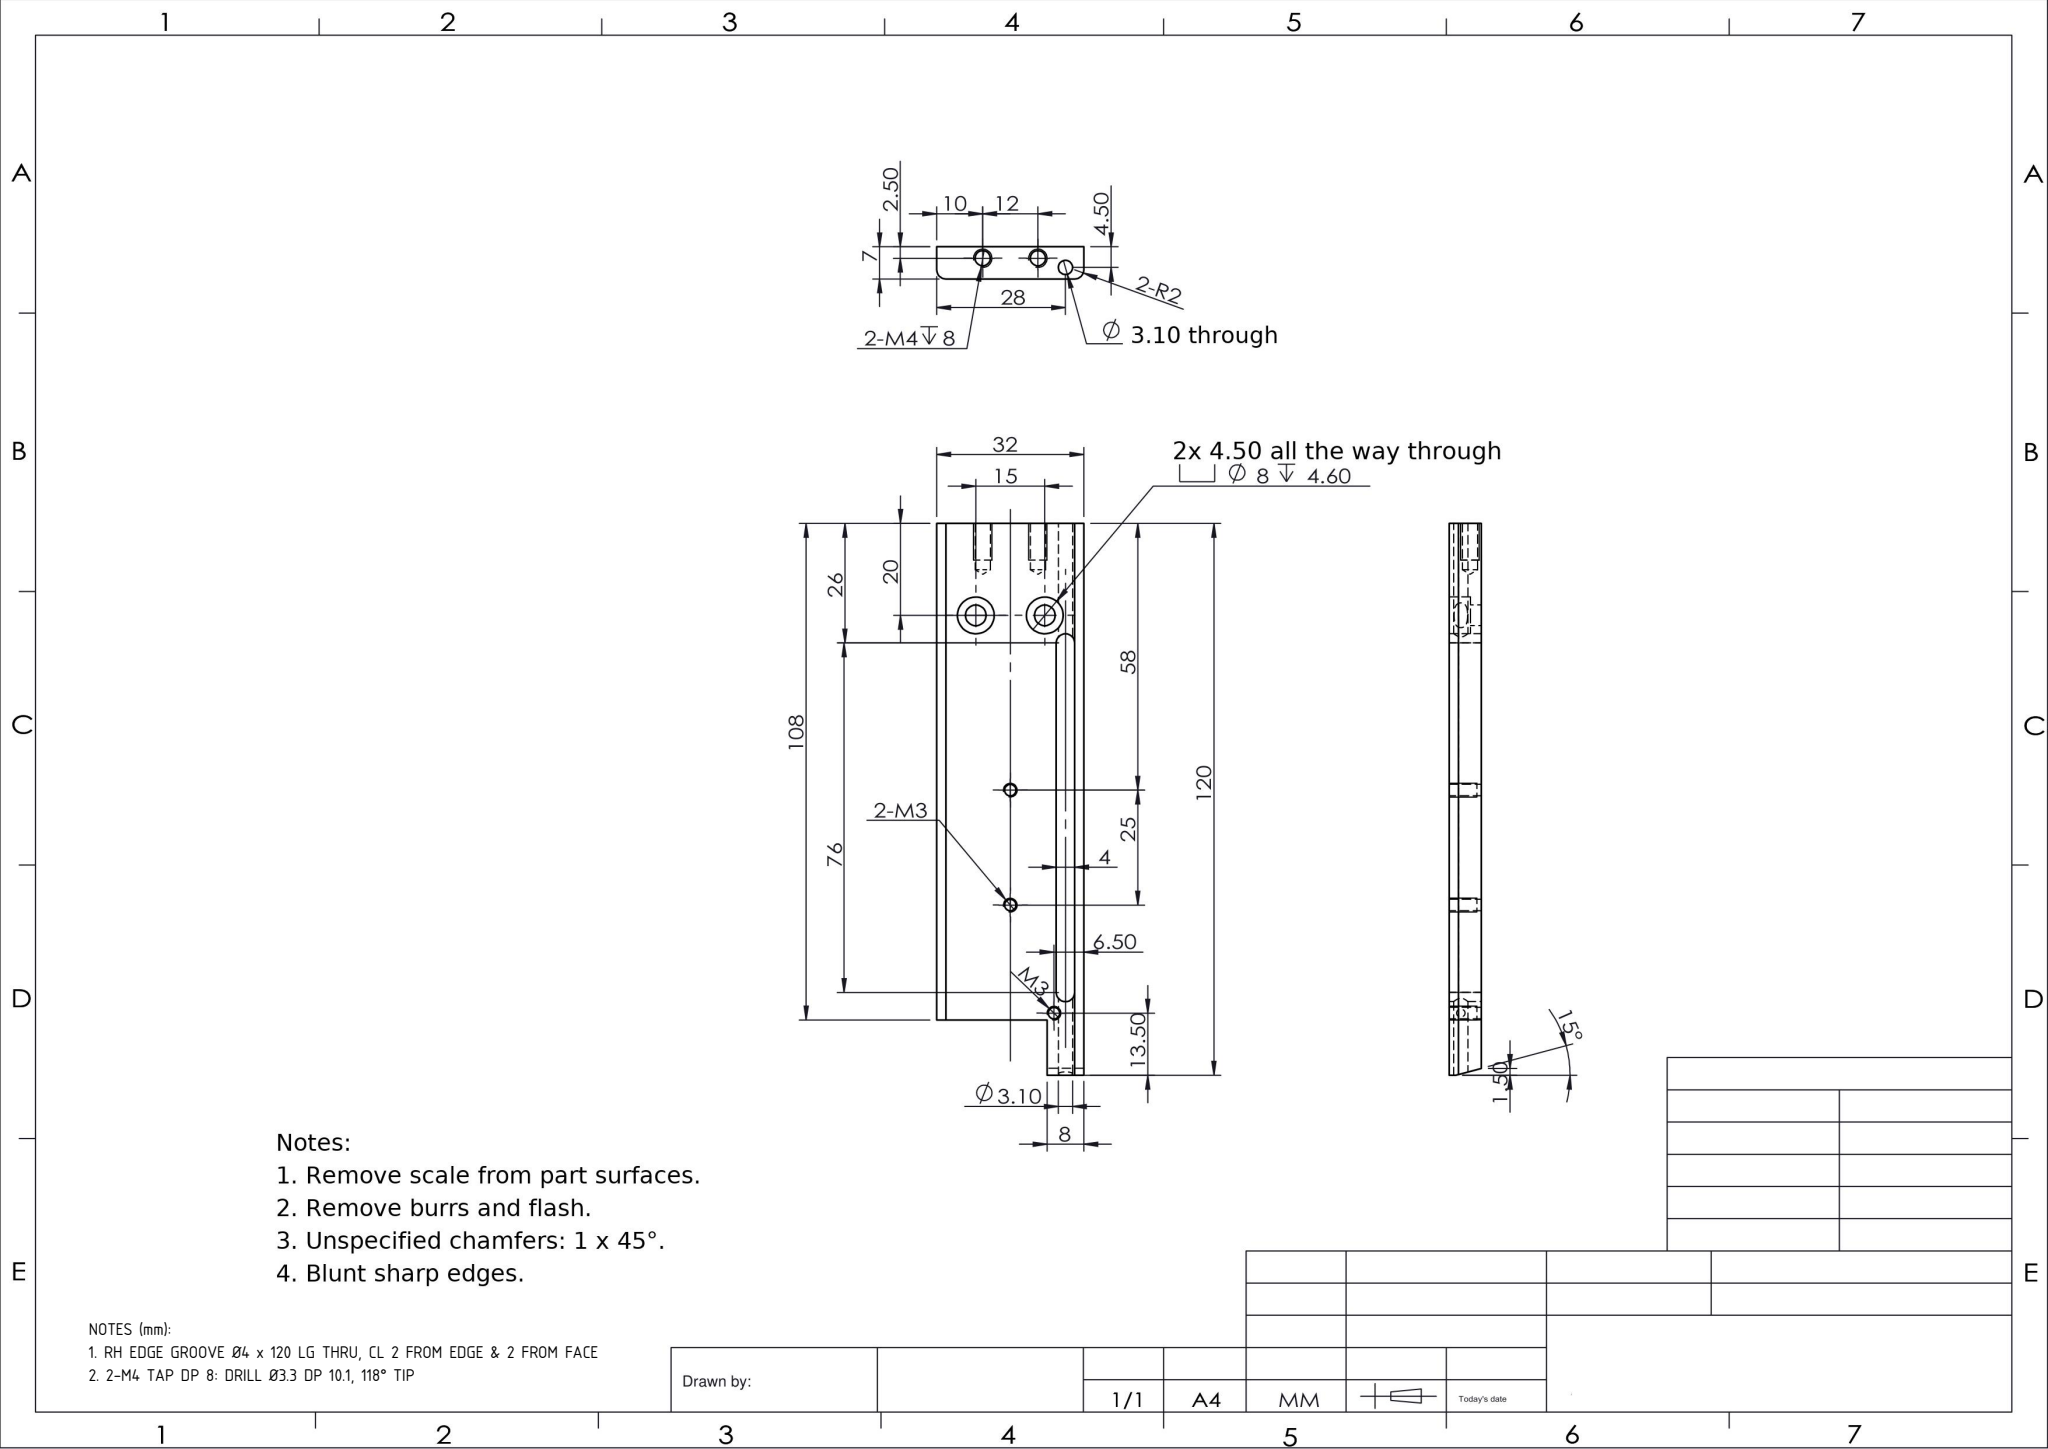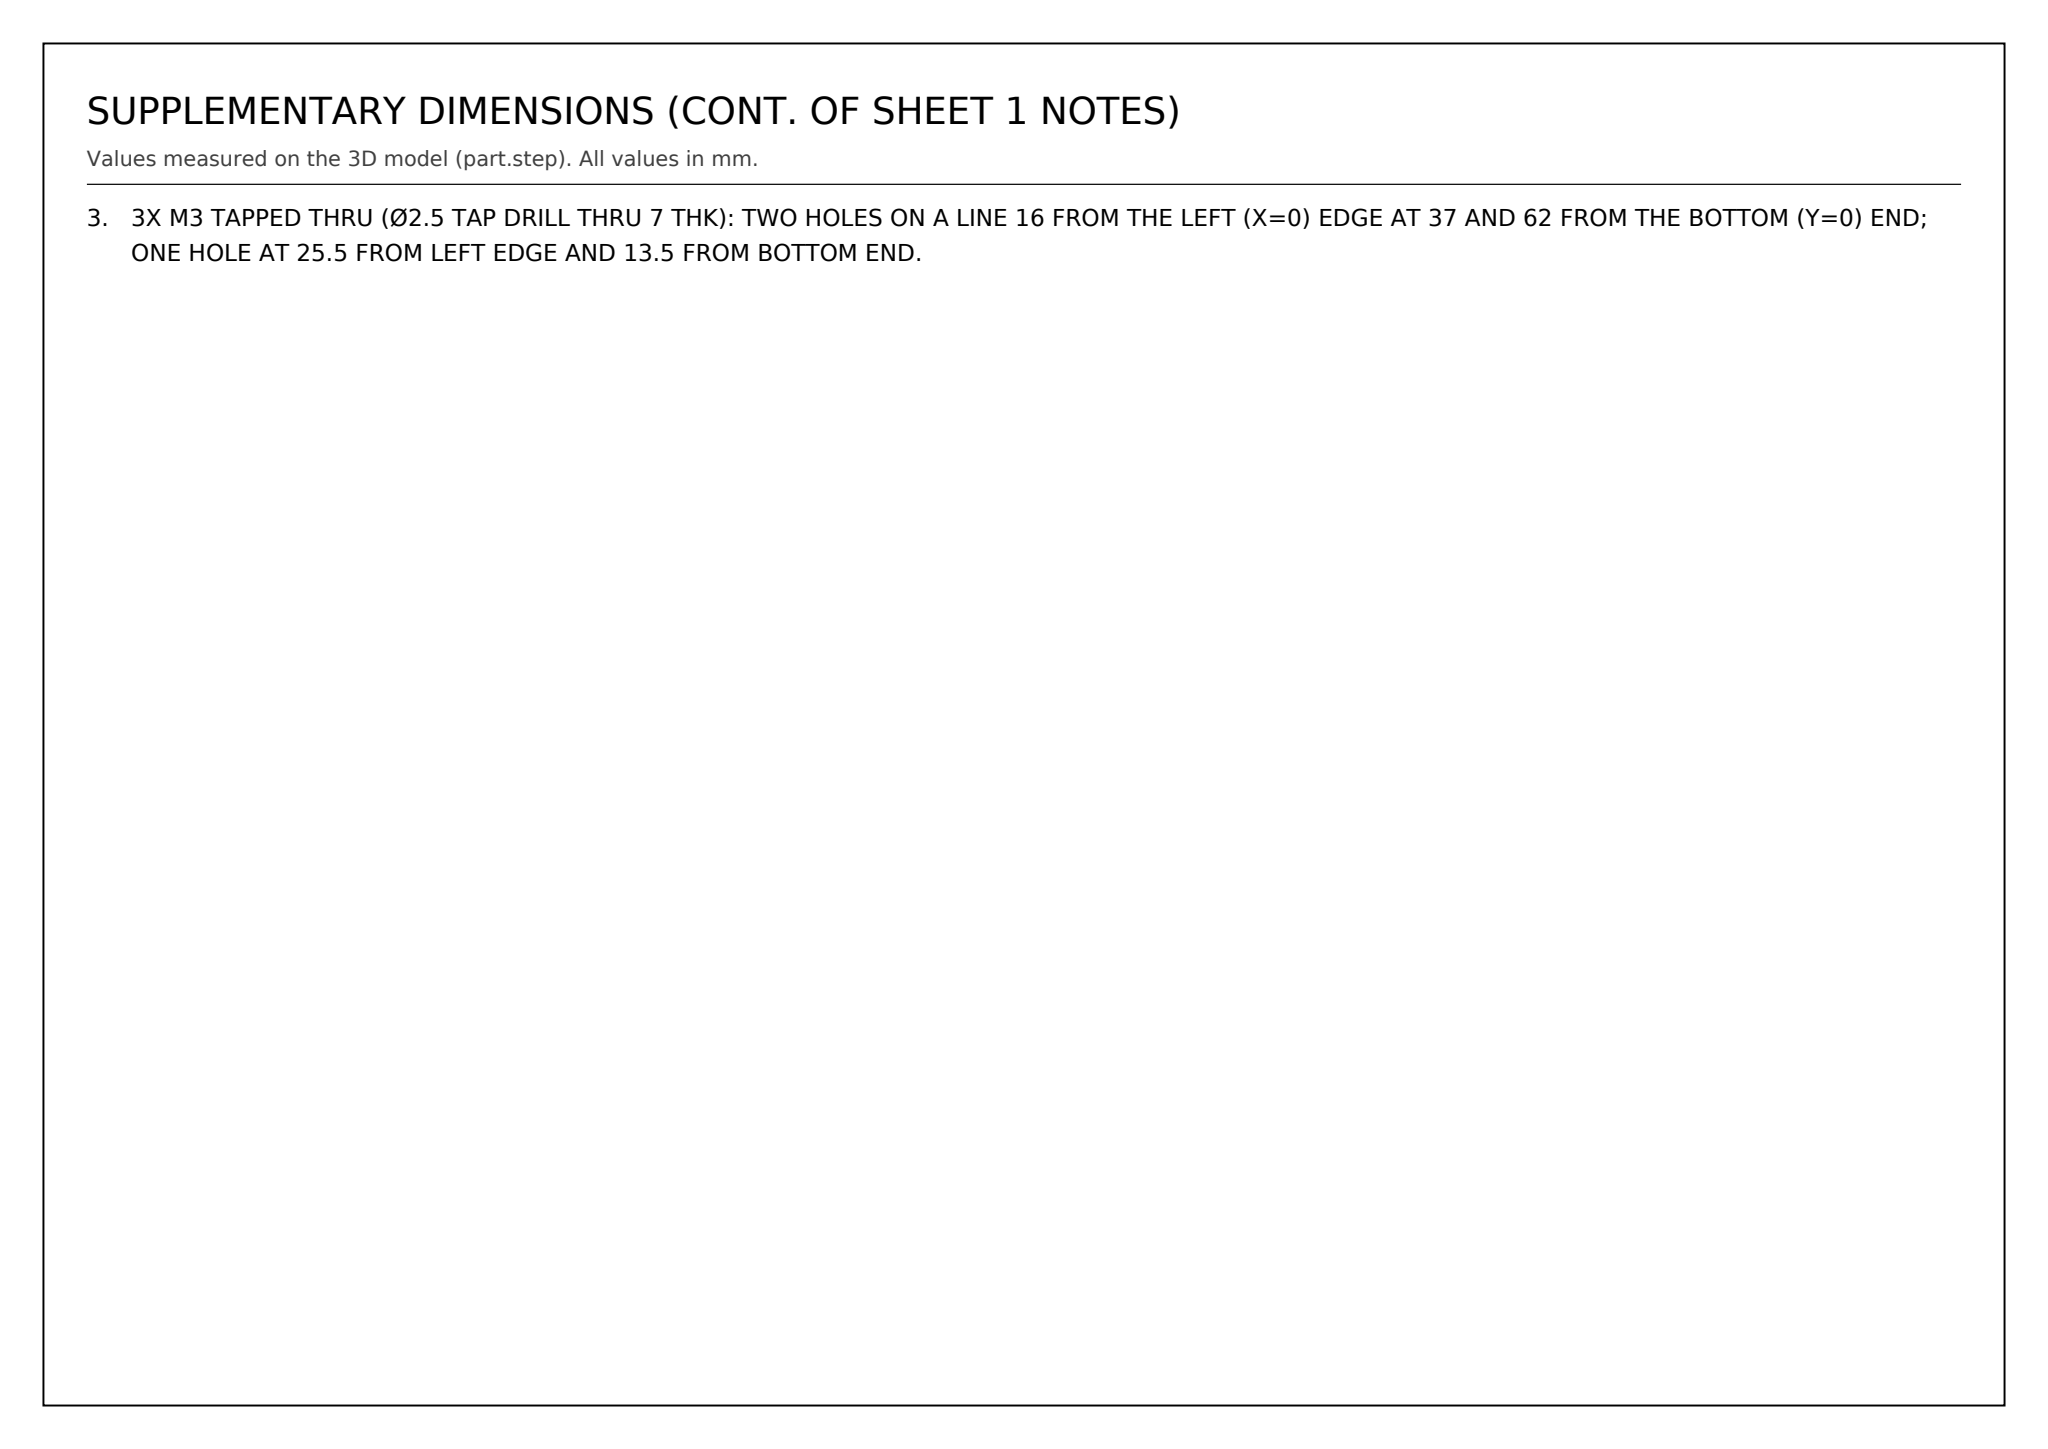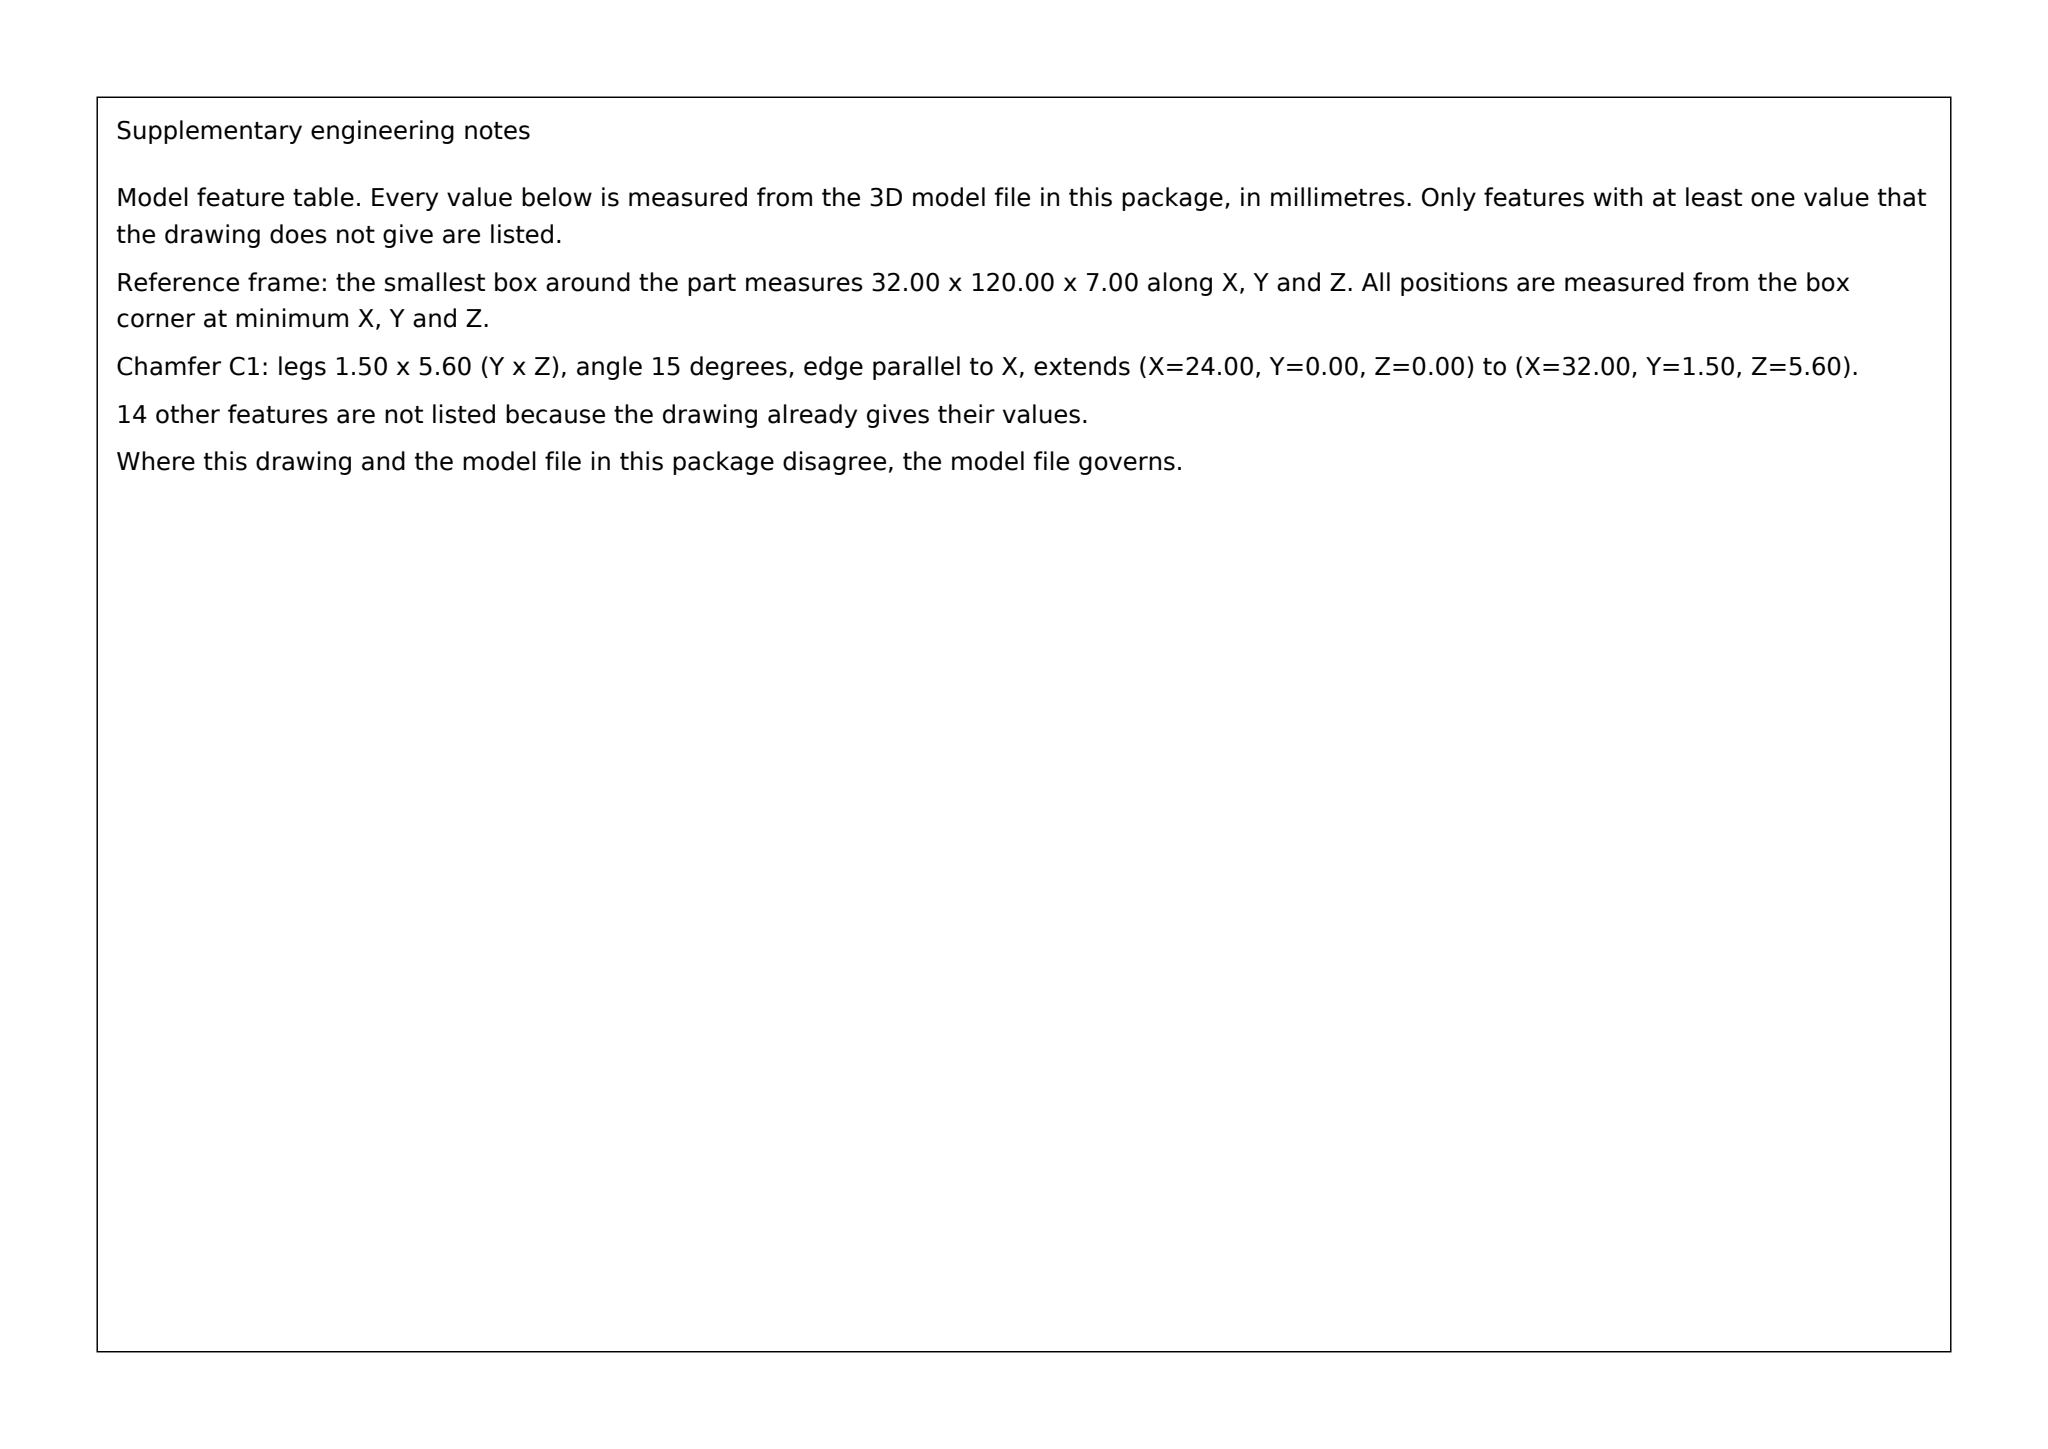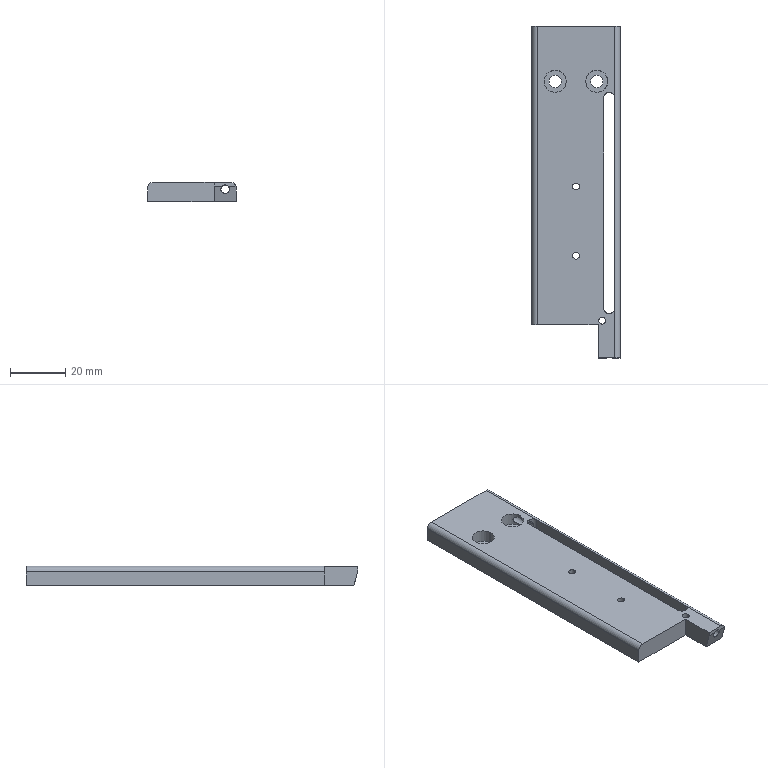Part | SolidWorks | mm | 1 solid | 45 faces | box 32 x 120 x 7 mm | volume 21304 mm3 | cylinder 28 | plane 13 | cone 4 | commonest cylinder face diameters 2.5 x6 4 x6 8 x4 4.5 x4 3.1 x4 3.3 x4
Drawing notes:
RH EDGE GROOVE Ø4 x 120 LG THRU, CL 2 FROM EDGE & 2 FROM FACE | from the solid: cyl Ø4 axis y at x=30, z=5, len 120; bbox x=32 (edge), z=7 (face) -> CL 2 from each
2-M4 TAP DP 8: DRILL Ø3.3 DP 10.1, 118° TIP | from the solid: cyl Ø3.3 axis y at x=10 & x=22, z=2.5, len 10.1 with 118° tip cone; matches top-view 2-M4↧8
3X M3 TAPPED THRU (Ø2.5 TAP DRILL THRU 7 THK): TWO HOLES ON A LINE 16 FROM THE LEFT (X=0) EDGE AT 37 AND 62 FROM THE BOTTOM (Y=0) END; ONE HOLE AT 25.5 FROM LEFT EDGE AND 13.5 FROM BOTTOM END. | from the solid: cylinders[hole/bore, dia 2.5, axis z] at (16,37), (16,62), (25.5,13.5), from z=0 to z=7 = full 7 mm plate thickness (bbox_xyz z=7)